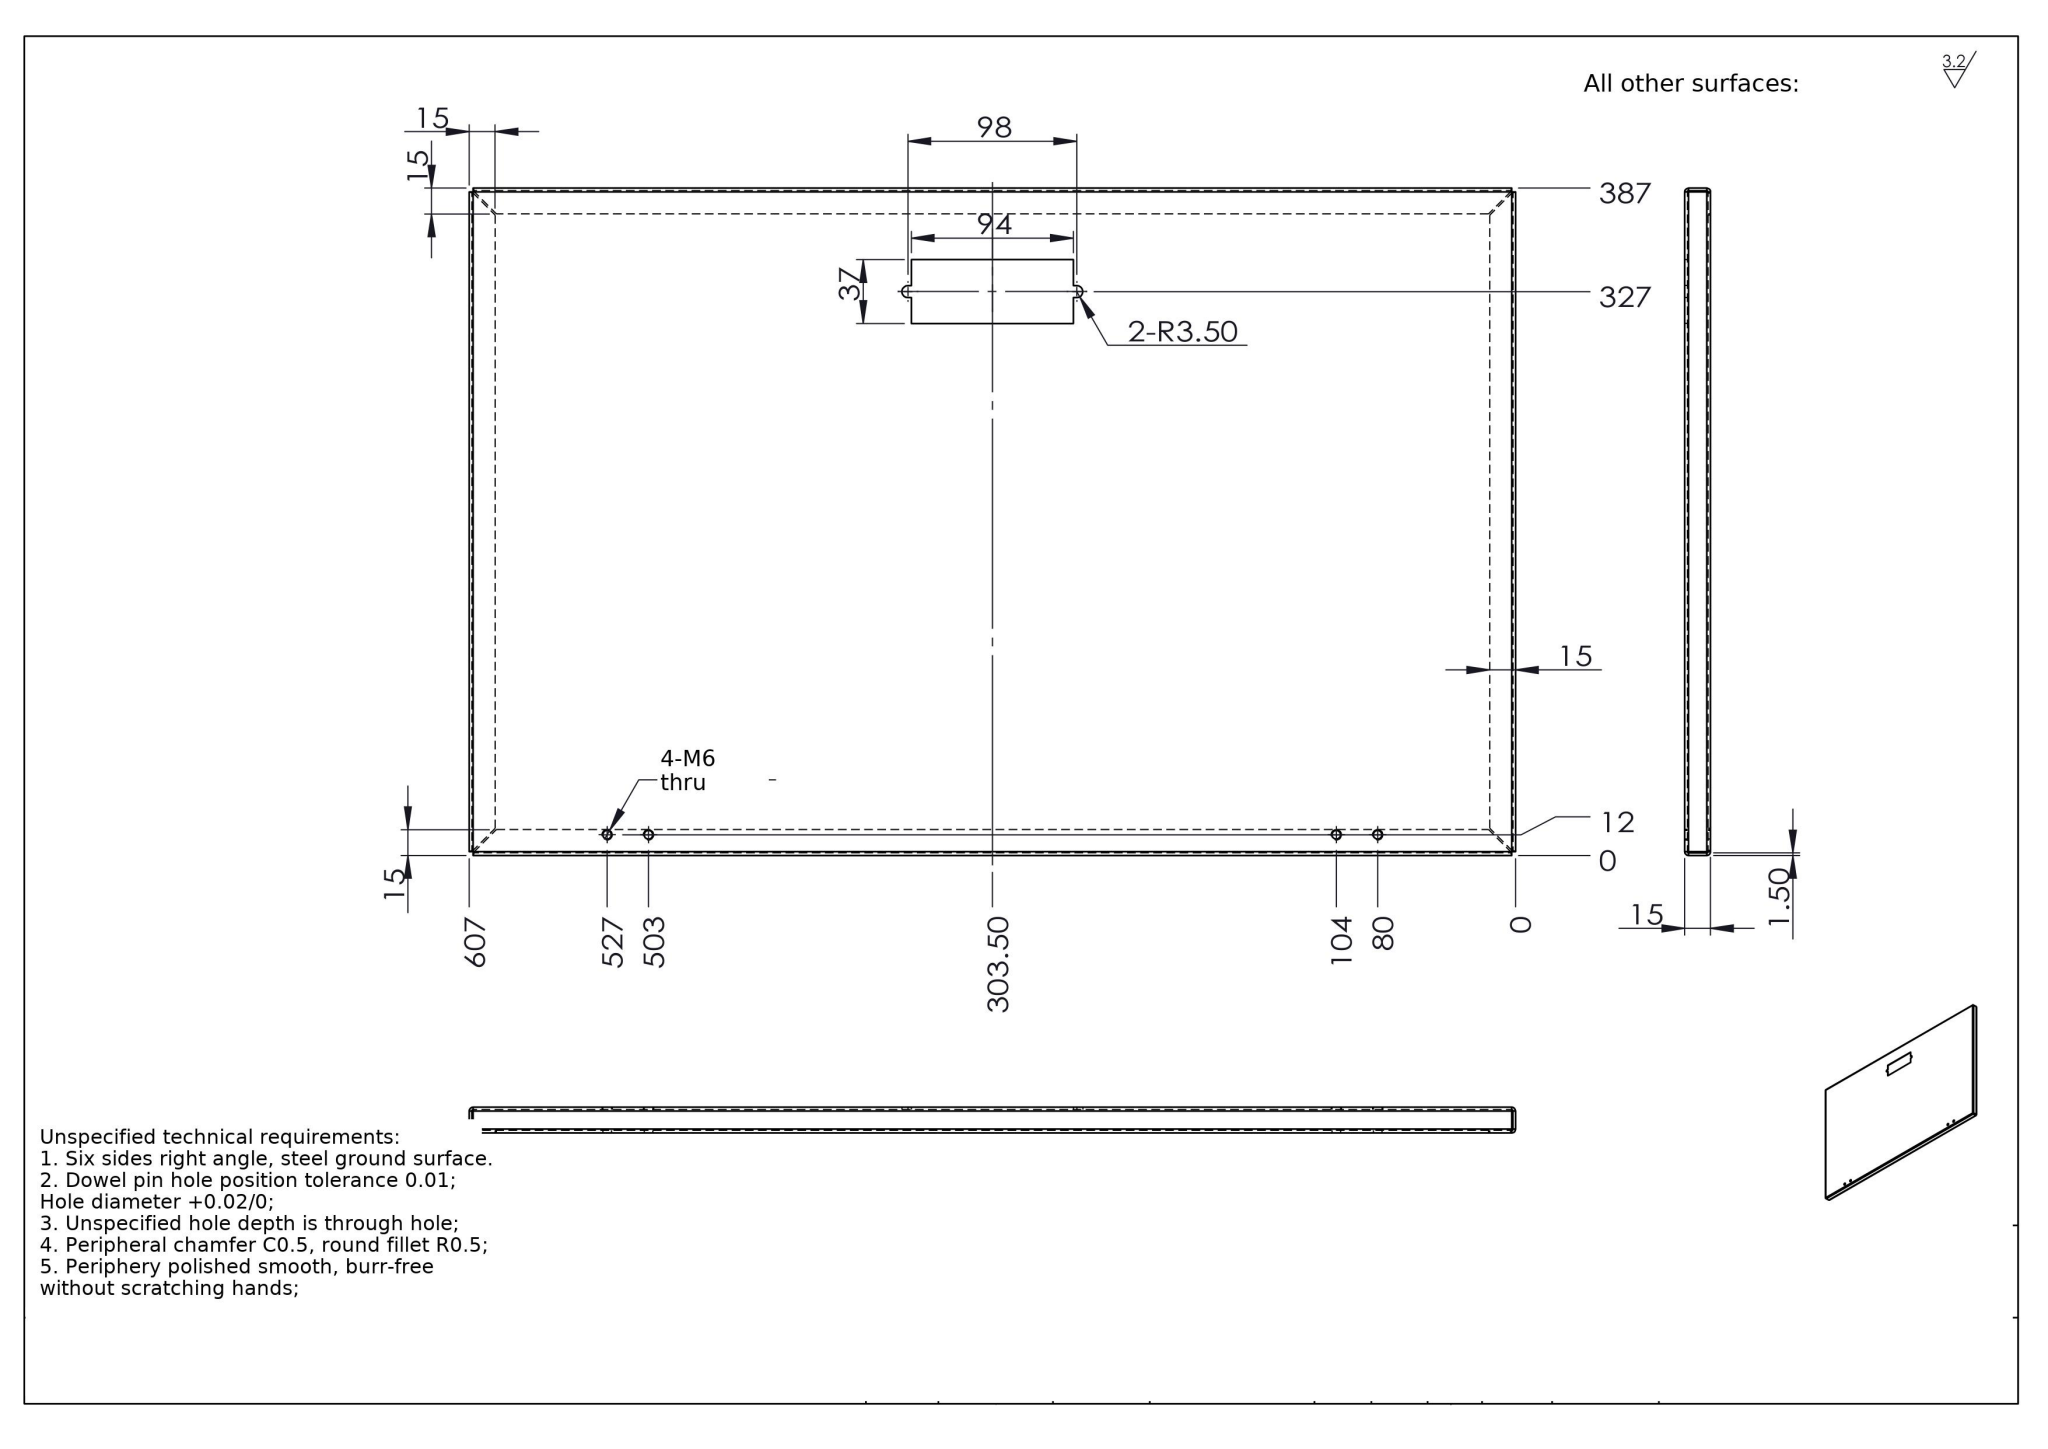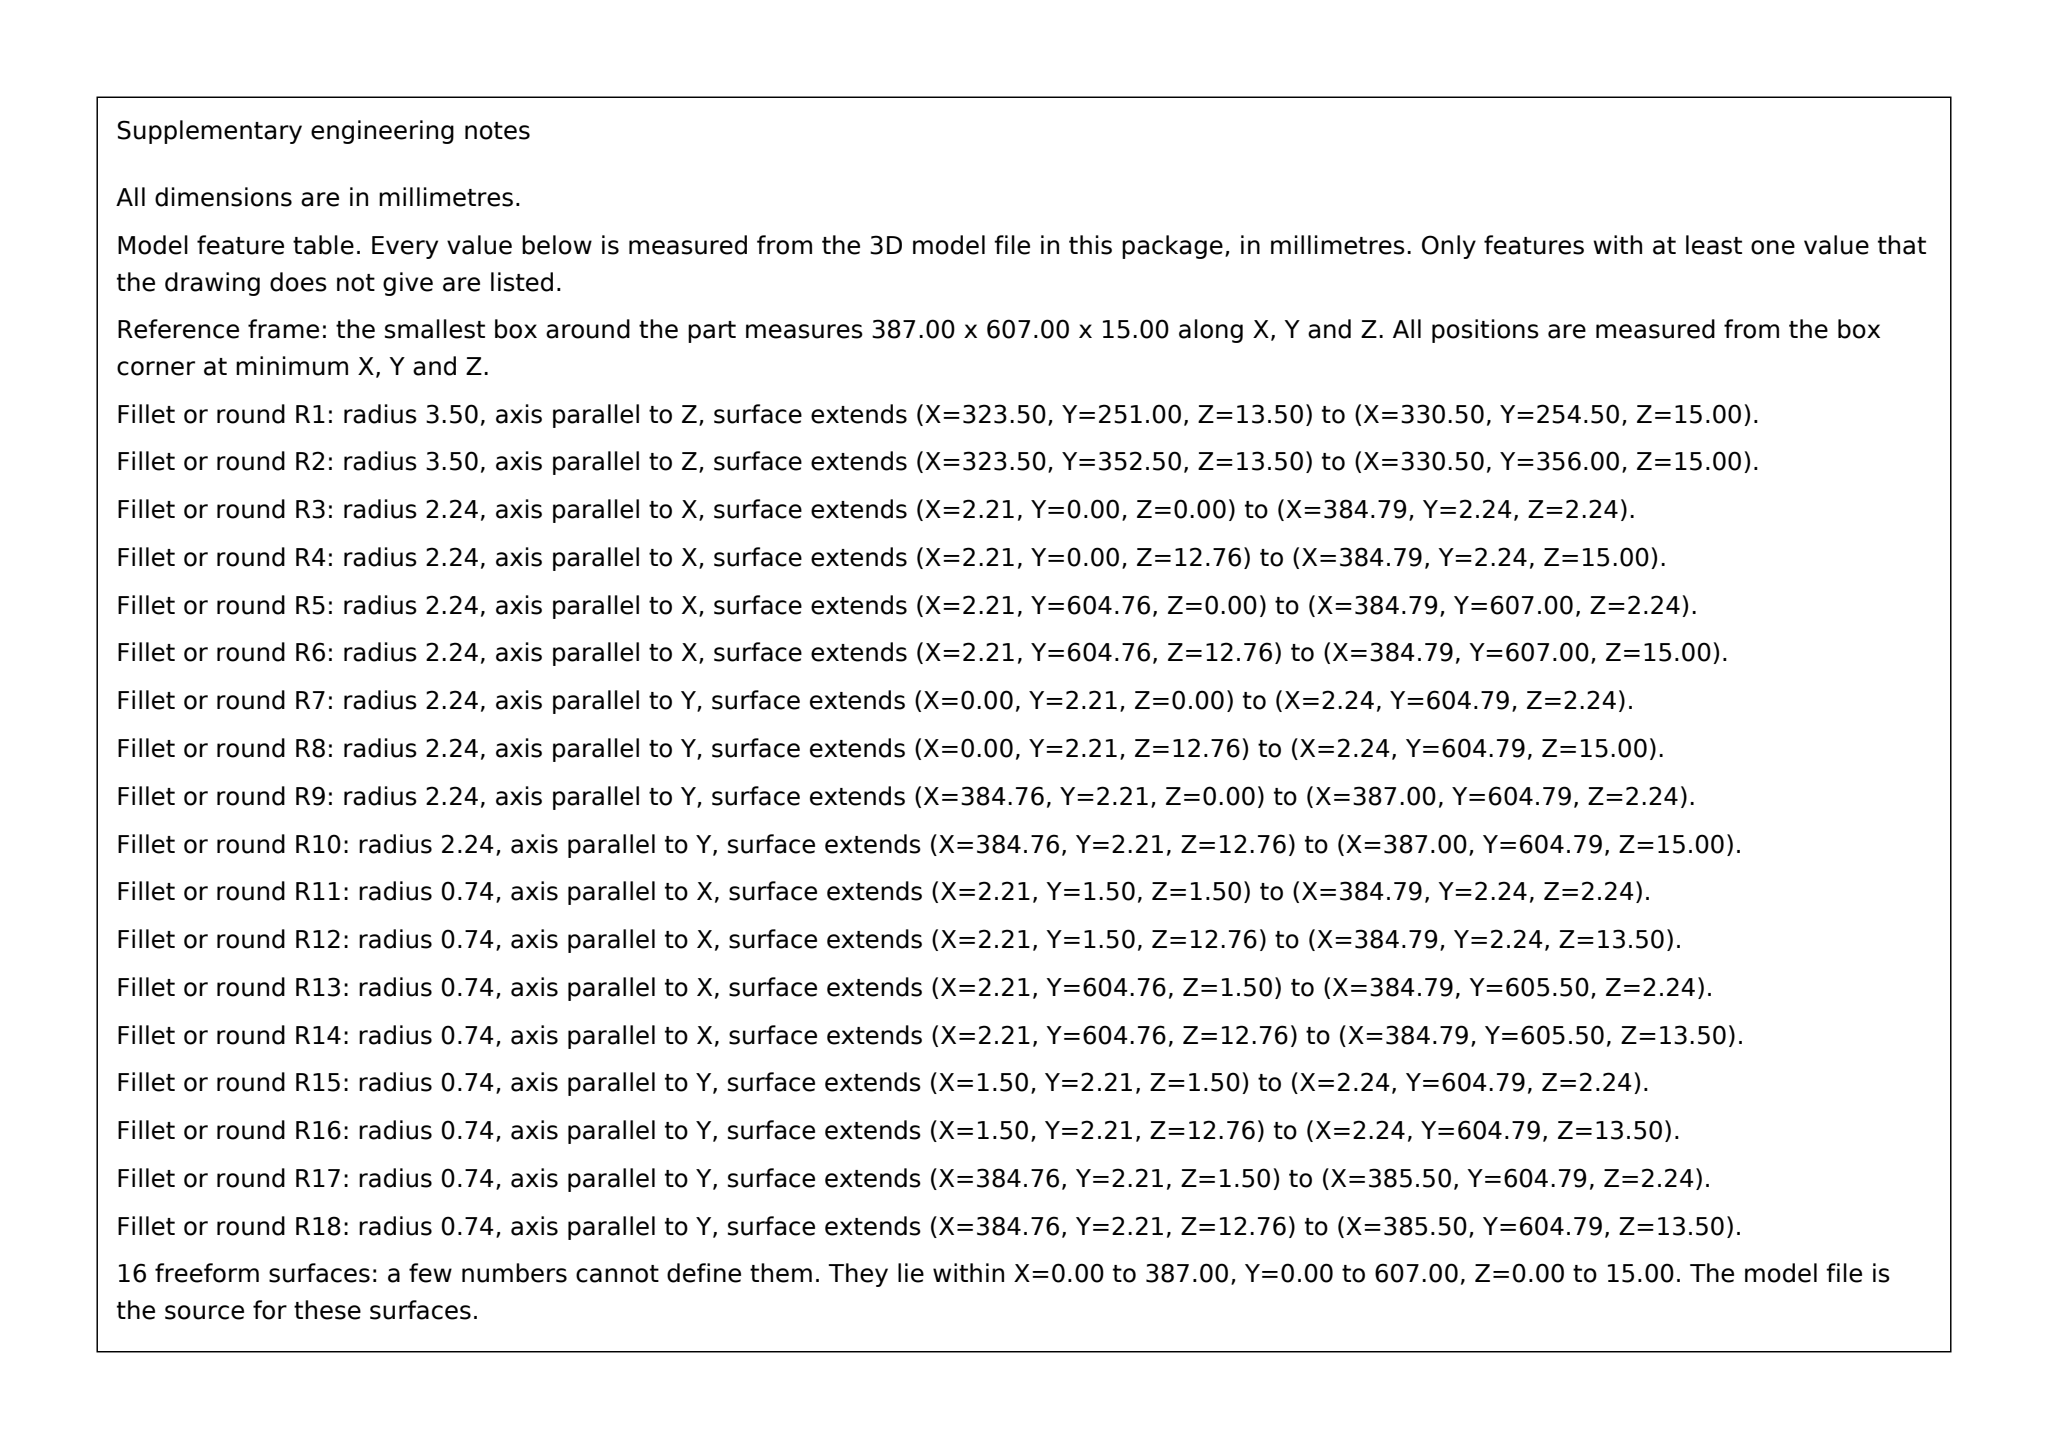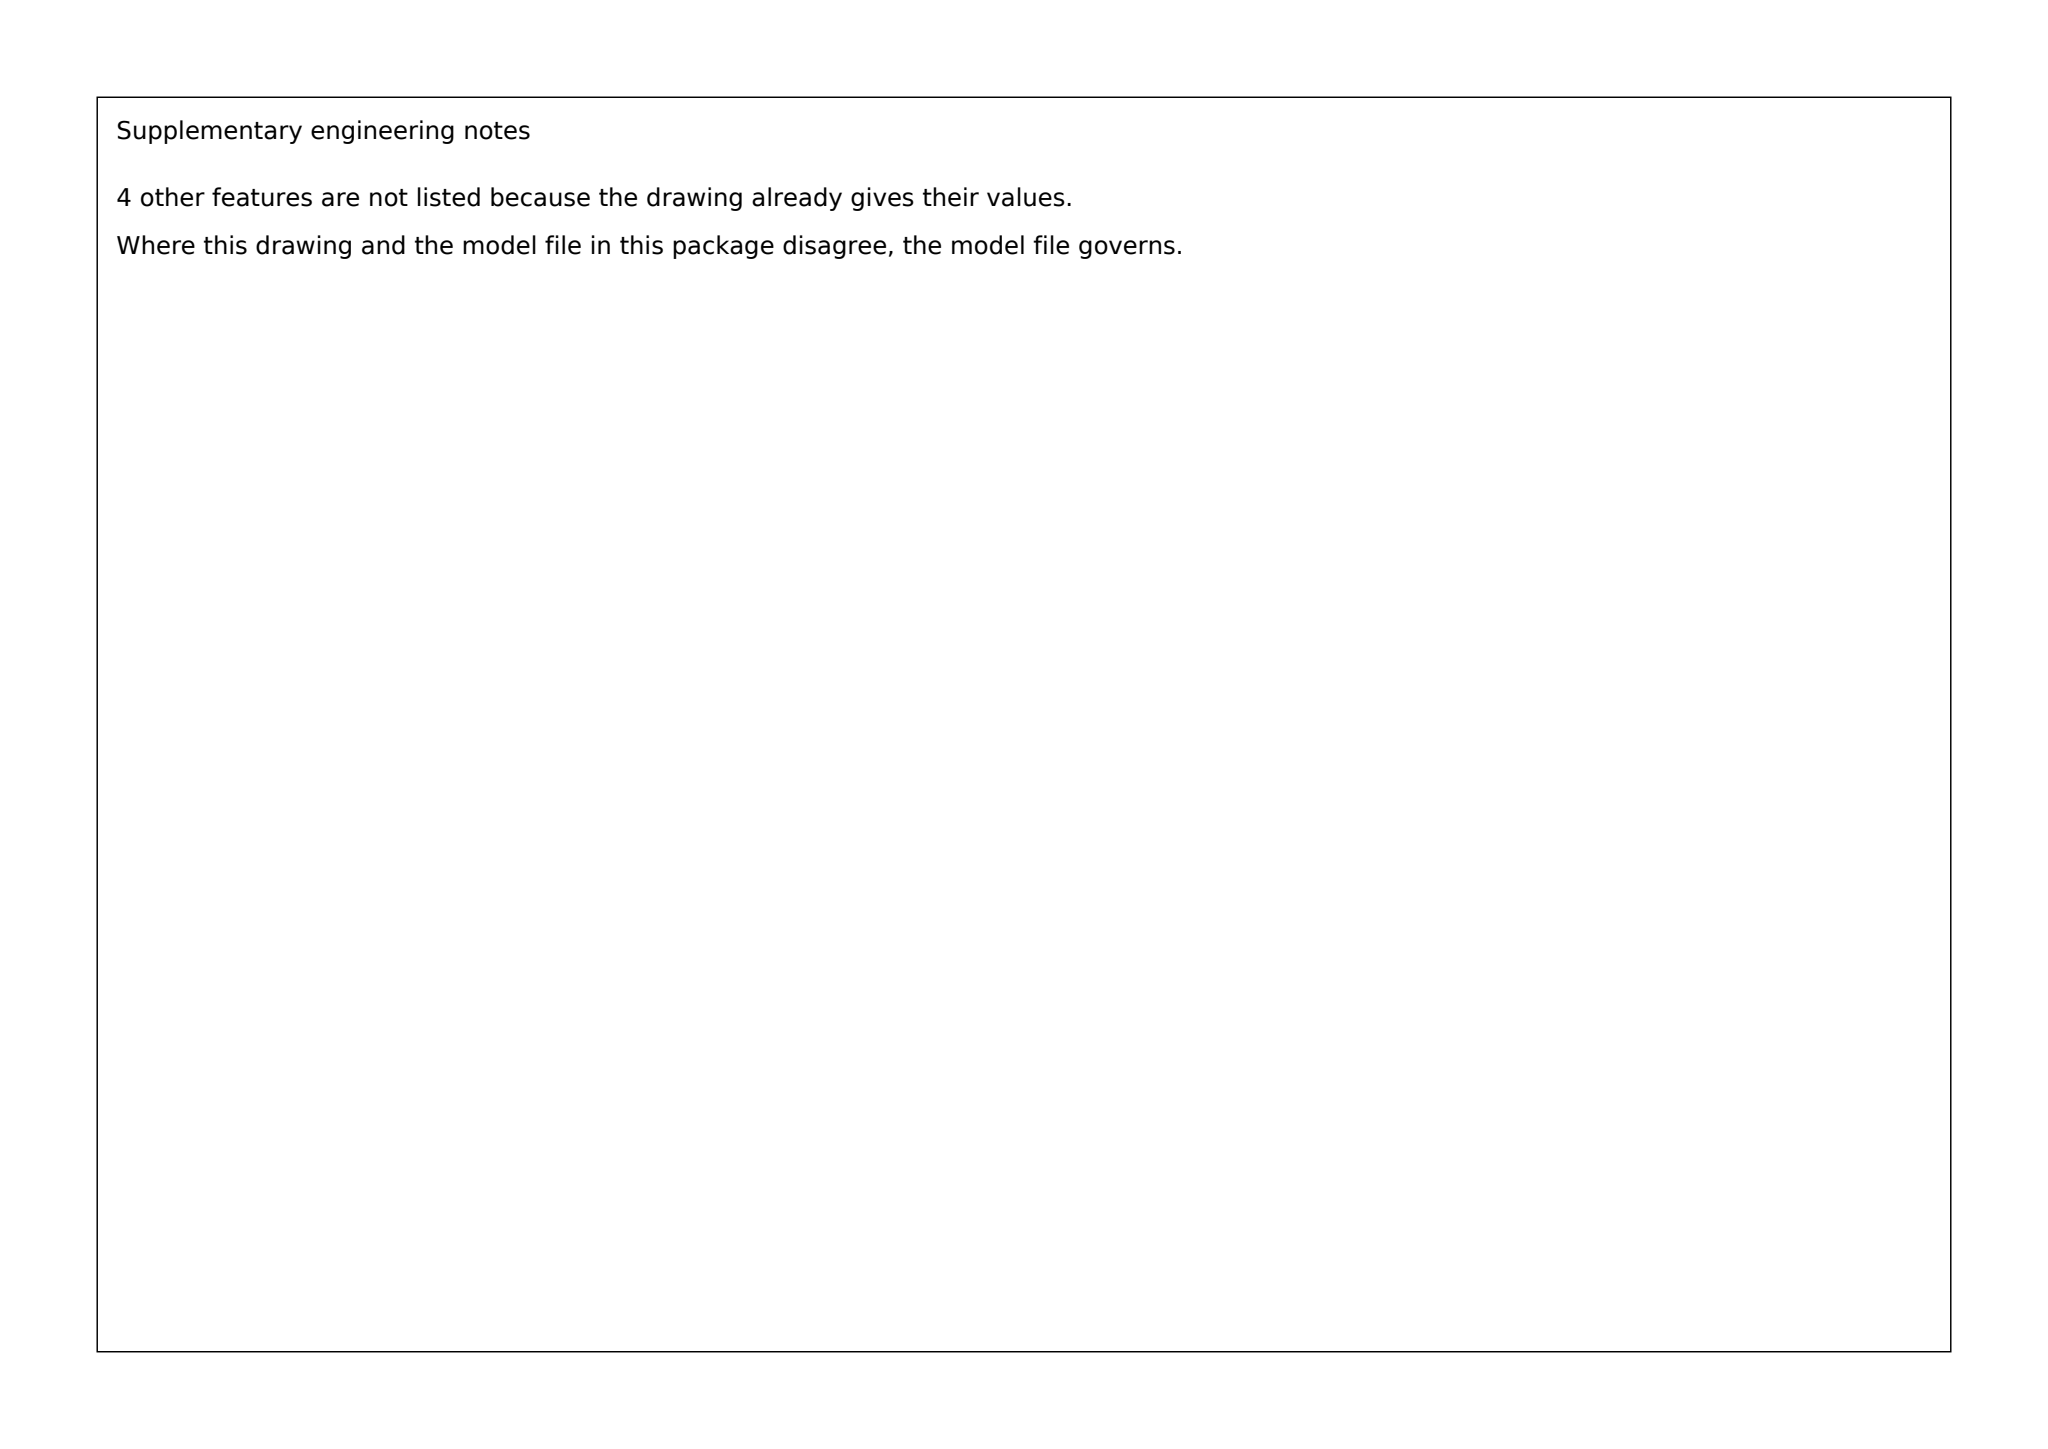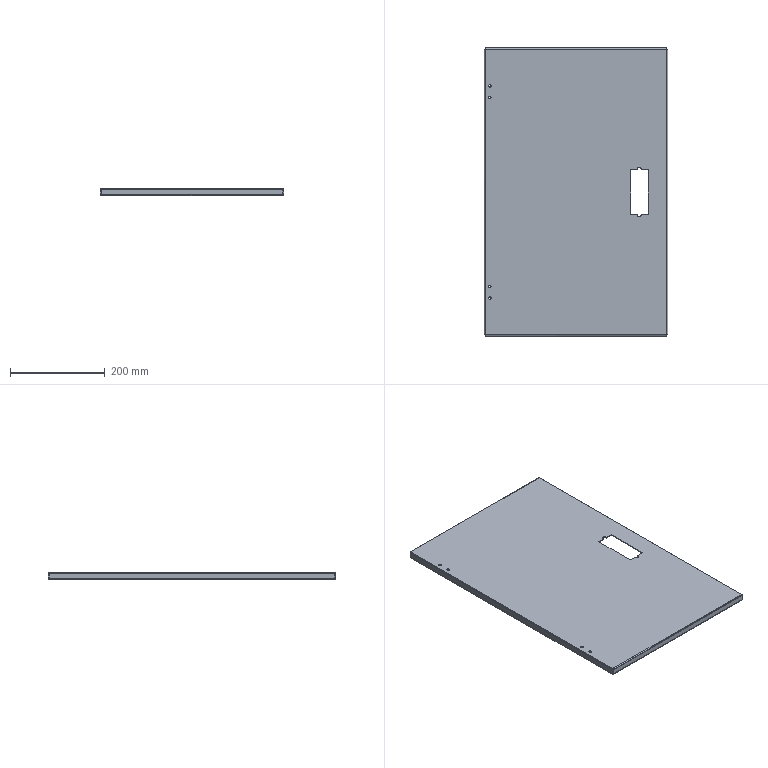Part | SolidWorks | mm | 1 solid | 98 faces | box 387 x 607 x 15 mm | volume 421708 mm3 | plane 48 | cylinder 34 | spline 16 | commonest cylinder face diameters 5 x16 4.473 x8 1.473 x8 7 x2